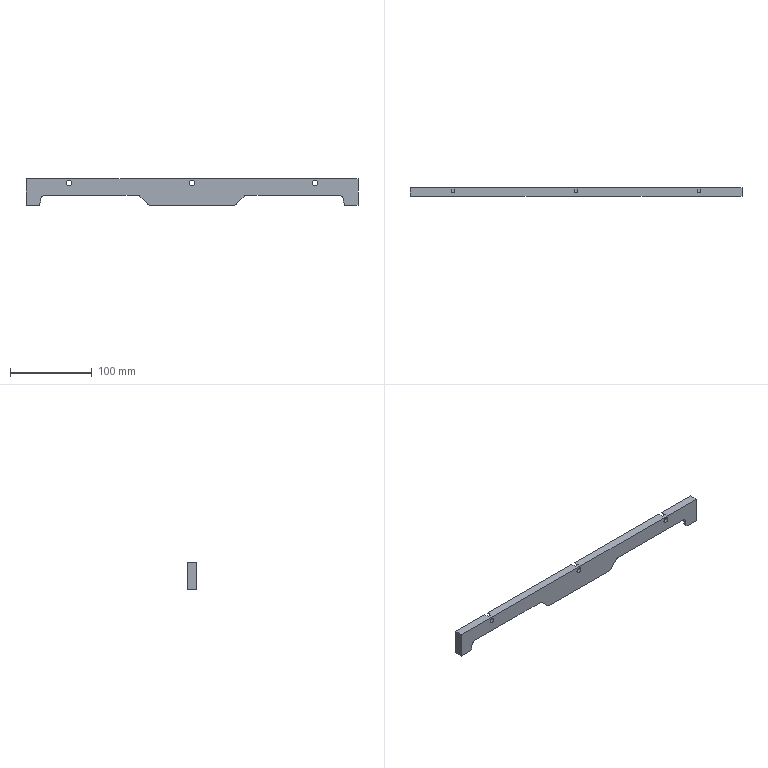Component | SolidWorks | 30-32A-1 | 1 solid | 55 faces | box 405 x 10 x 32 mm | volume 74300 mm3 | plane 32 | cylinder 17 | cone 6 | commonest cylinder face diameters 10 x8 6.6 x6 11 x3
build123d program:
from build123d import *
from OCP.BRepFilletAPI import BRepFilletAPI_MakeChamfer

# Parameters (mm, degrees)
SKETCH1_W                                            = 405
SKETCH1_H                                            = 10
EXTRUDE1_DEPTH                                       = 20
CUT_EXTRUDE12_DEPTH                                  = 6
EXTRUDE2_DEPTH                                       = 4
EXTRUDE3_DEPTH                                       = 12
COUNTERBORE_FOR_M6_HEXAGON_SOCKET_HEAD_C_D           = 6.6
COUNTERBORE_FOR_M6_HEXAGON_SOCKET_HEAD_C_CBORE_D     = 11
COUNTERBORE_FOR_M6_HEXAGON_SOCKET_HEAD_C_CBORE_DEPTH = 6
FILLET1_R                                            = 5
CHAMFER4_SIZE                                        = 0.5
CHAMFER5_SIZE                                        = 2
CHAMFER5_SIZE2                                       = 3.464


with BuildPart() as part:
    # Sketch1 → Extrude1 (new body)
    with BuildSketch(Plane.XY):
        Rectangle(SKETCH1_W, SKETCH1_H)
    extrude(amount=EXTRUDE1_DEPTH)

    # Sketch26 → Cut-Extrude12 (cut)
    with BuildSketch(Plane(origin=(0, 5, 0), x_dir=(1, 0, 0), z_dir=(0, 1, 0))):
        with BuildLine():
            Line((190.5, 0), (190.5, -1))
            ThreePointArc((190.5, -1), (189.036, -4.536), (185.5, -6))
            Line((185.5, -6), (-185.5, -6))
            ThreePointArc((-185.5, -6), (-189.036, -4.536), (-190.5, -1))
            Line((-190.5, -1), (-190.5, 0))
            Line((-190.5, 0), (190.5, 0))
        make_face()
    extrude(amount=-CUT_EXTRUDE12_DEPTH, mode=Mode.SUBTRACT)

    # Sketch31 → Extrude2 (add)
    with BuildSketch(Plane(origin=(0, -1, 0), x_dir=(1, 0, 0), z_dir=(0, 1, 0))):
        Polygon((-65, 0), (-53, 12), (53, 12), (65, 0), align=None)
    extrude(amount=-EXTRUDE2_DEPTH)

    # Sketch32 → Extrude3 (add)
    with BuildSketch(Plane(origin=(0, 0, 0), x_dir=(-1, 0, 0), z_dir=(0, 0, -1))):
        Polygon((-202.5, 5), (-190.5, 5), (-190.5, -1), (-184.5, -1), (-184.5, -5), (-202.5, -5), align=None)
        Polygon((184.5, -1), (184.5, -5), (202.5, -5), (202.5, 5), (190.5, 5), (190.5, -1), align=None)
    extrude(amount=EXTRUDE3_DEPTH)

    # Counterbore for M6 Hexagon Socket Head C (through all)
    with Locations(Plane(origin=(0, 5, 0), x_dir=(-1, 0, 0), z_dir=(0, 1, 0))):
        with Locations((150, 15), (0, 15), (-150, 15)):
            CounterBoreHole(COUNTERBORE_FOR_M6_HEXAGON_SOCKET_HEAD_C_D / 2, COUNTERBORE_FOR_M6_HEXAGON_SOCKET_HEAD_C_CBORE_D / 2, COUNTERBORE_FOR_M6_HEXAGON_SOCKET_HEAD_C_CBORE_DEPTH)

    # Fillet1
    fillet1_edges = [part.edges().sort_by_distance(p)[0] for p in [
        (-65, -3, 0),
        (-53, -3, -12),
        (53, -3, -12),
        (65, -3, 0),
        (184.5, -3, 0),
        (-184.5, -3, 0),
    ]]
    fillet(fillet1_edges, radius=FILLET1_R)

    # Chamfer4
    chamfer4_edges = [part.edges().sort_by_distance(p)[0] for p in [
        (-123.286, -1, 0),
        (123.286, -1, 0),
        (-59, -1, -6),
        (0, -1, -12),
        (59, -1, -6),
        (52.842, -1, -11.619),
        (-52.842, -1, -11.619),
        (-183.036, -1, -1.464),
        (183.036, -1, -1.464),
        (-65.158, -1, -0.3806),
        (65.158, -1, -0.3806),
        (184.5, -1, -8.5),
        (-184.5, -1, -8.5),
    ]]
    chamfer(chamfer4_edges, length=CHAMFER4_SIZE)

    # Chamfer5: one chamfer whose edges measure the first distance from different faces: ONE call of the kernel's chamfer builder (chamfer() names one face for all edges)
    chamfer5_edges_1 = [part.edges().sort_by_distance(p)[0] for p in [
        (190.5, 2, -12),
        (184.5, -3.25, -12),
    ]]
    chamfer5_side_1 = [part.faces().sort_by_distance(p)[0] for p in [
        (195.009, -0.4994, -12),
    ]]
    chamfer5_edges_2 = [part.edges().sort_by_distance(p)[0] for p in [
        (-184.5, -3.25, -12),
        (-190.5, 2, -12),
    ]]
    chamfer5_side_2 = [part.faces().sort_by_distance(p)[0] for p in [
        (-195.009, -0.4994, -12),
    ]]
    chamfer5 = BRepFilletAPI_MakeChamfer(part.part.solid().wrapped)
    for e in chamfer5_edges_1:
        chamfer5.Add(CHAMFER5_SIZE, CHAMFER5_SIZE2, e.wrapped, chamfer5_side_1[0].wrapped)  # the first distance lies on this face
    for e in chamfer5_edges_2:
        chamfer5.Add(CHAMFER5_SIZE, CHAMFER5_SIZE2, e.wrapped, chamfer5_side_2[0].wrapped)  # the first distance lies on this face
    add(Compound.cast(chamfer5.Shape()), mode=Mode.REPLACE)


solid = part.part

# Placed as in the assembly
solid = solid.moved(Location((-649.208, 21.908, 709.188), (0, 0, 0)))